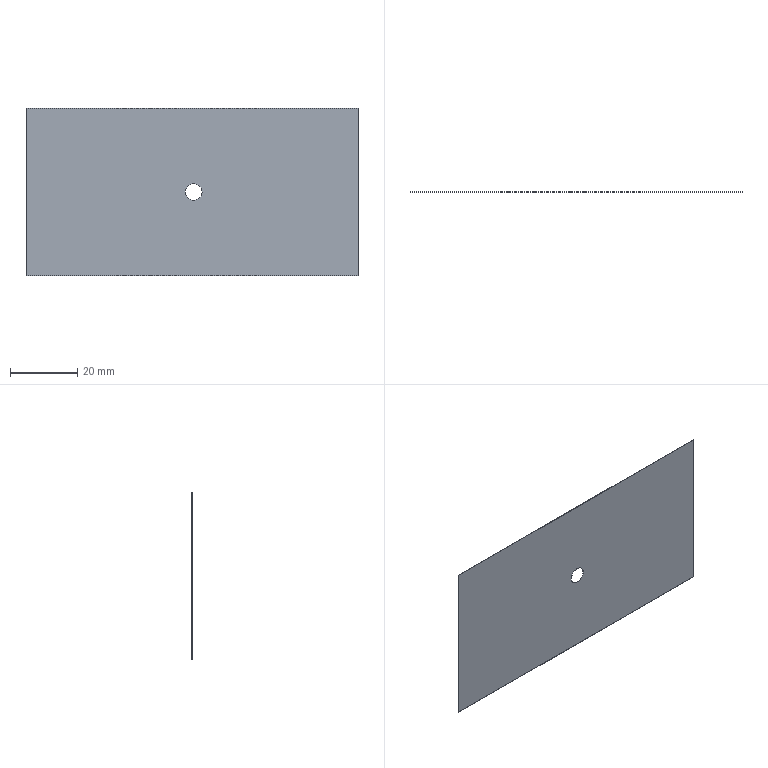Component | SolidWorks | WashingLabel100-50-1 | 1 solid | 8 faces | box 99 x 0.1 x 50 mm | volume 493 mm3 | plane 6 | cylinder 2 | commonest cylinder face diameters 5 x2 | material Zoltek Panex 33
build123d program:
from build123d import *

# Parameters (mm, degrees)
SKETCH1_W           = 50
SKETCH1_H           = 100
BOSS_EXTRUDE1_DEPTH = 0.1
SKETCH2_R           = 2.5
CUT_EXTRUDE1_DEPTH  = 10
BENDRADIUSRELIEF_BY = 1


with BuildPart() as part:
    # Sketch1 → Boss-Extrude1 (new body)
    with BuildSketch(Plane(origin=(0, 0, 0), x_dir=(1, 0, 0), z_dir=(0, 1, 0))):
        Rectangle(SKETCH1_W, SKETCH1_H)
    extrude(amount=BOSS_EXTRUDE1_DEPTH)

    # Sketch2 → Cut-Extrude1 (cut)
    with BuildSketch(Plane(origin=(0, 0.1, 0), x_dir=(1, 0, 0), z_dir=(0, 1, 0))):
        with Locations(Location((0, 0, 0), (0, 0, 270))):
            Circle(SKETCH2_R)
    extrude(amount=-CUT_EXTRUDE1_DEPTH, mode=Mode.SUBTRACT)

    # BendRadiusRelief: a face moved inward by 1.0
    extrude(part.faces().sort_by_distance((0, 0.05, -50))[0], amount=BENDRADIUSRELIEF_BY, dir=(0, 0, 1), mode=Mode.SUBTRACT)


solid = part.part

# Placed as in the assembly
solid = solid.moved(Location((12, 0, 0), (0, -90, 0)))
STEP:
#1=COLOUR_RGB('',0.7922,0.8196,0.9333);
#2=FILL_AREA_STYLE_COLOUR('',#1);
#3=FILL_AREA_STYLE('',(#2));
#4=SURFACE_STYLE_FILL_AREA(#3);
#5=SURFACE_SIDE_STYLE('',(#4));
#6=SURFACE_STYLE_USAGE(.BOTH.,#5);
#7=PRESENTATION_STYLE_ASSIGNMENT((#6));
#8=CARTESIAN_POINT('',(0.5709,0.,-0.));
#9=VERTEX_POINT('',#8);
#10=CARTESIAN_POINT('',(0.374,0.,-0.));
#11=VERTEX_POINT('',#10);
#12=CARTESIAN_POINT('',(0.4724,0.,-0.));
#13=DIRECTION('',(0.,1.,0.));
#14=DIRECTION('',(-1.,0.,-0.));
#15=AXIS2_PLACEMENT_3D('',#12,#13,#14);
#16=CIRCLE('',#15,0.09843);
#17=EDGE_CURVE('',#9,#11,#16,.T.);
#18=ORIENTED_EDGE('',*,*,#17,.F.);
#19=CARTESIAN_POINT('',(0.5709,0.003937,-0.));
#20=VERTEX_POINT('',#19);
#21=CARTESIAN_POINT('',(0.5709,-0.3898,-0.));
#22=DIRECTION('',(0.,1.,0.));
#23=VECTOR('',#22,39.37);
#24=LINE('',#21,#23);
#25=EDGE_CURVE('',#9,#20,#24,.T.);
#26=ORIENTED_EDGE('',*,*,#25,.T.);
#27=CARTESIAN_POINT('',(0.374,0.003937,-0.));
#28=VERTEX_POINT('',#27);
#29=CARTESIAN_POINT('',(0.4724,0.003937,-0.));
#30=DIRECTION('',(0.,1.,0.));
#31=DIRECTION('',(-1.,0.,-0.));
#32=AXIS2_PLACEMENT_3D('',#29,#30,#31);
#33=CIRCLE('',#32,0.09843);
#34=EDGE_CURVE('',#20,#28,#33,.T.);
#35=ORIENTED_EDGE('',*,*,#34,.T.);
#36=CARTESIAN_POINT('',(0.374,-0.3898,-0.));
#37=DIRECTION('',(0.,1.,0.));
#38=VECTOR('',#37,39.37);
#39=LINE('',#36,#38);
#40=EDGE_CURVE('',#11,#28,#39,.T.);
#41=ORIENTED_EDGE('',*,*,#40,.F.);
#42=EDGE_LOOP('',(#18,#26,#35,#41));
#43=FACE_OUTER_BOUND('',#42,.T.);
#44=CARTESIAN_POINT('',(0.4724,-0.3898,-0.));
#45=DIRECTION('',(0.,1.,0.));
#46=DIRECTION('',(-1.,0.,-0.));
#47=AXIS2_PLACEMENT_3D('',#44,#45,#46);
#48=CYLINDRICAL_SURFACE('',#47,0.09843);
#49=ADVANCED_FACE('',(#43),#48,.F.);
#50=CARTESIAN_POINT('',(-1.496,0.,0.9843));
#51=VERTEX_POINT('',#50);
#52=CARTESIAN_POINT('',(2.402,0.,0.9843));
#53=VERTEX_POINT('',#52);
#54=CARTESIAN_POINT('',(2.441,0.,0.9843));
#55=DIRECTION('',(1.,-0.,-0.));
#56=VECTOR('',#55,39.37);
#57=LINE('',#54,#56);
#58=EDGE_CURVE('',#51,#53,#57,.T.);
#59=ORIENTED_EDGE('',*,*,#58,.T.);
#60=CARTESIAN_POINT('',(2.402,0.003937,0.9843));
#61=VERTEX_POINT('',#60);
#62=CARTESIAN_POINT('',(2.402,0.003937,0.9843));
#63=DIRECTION('',(-0.,-1.,-0.));
#64=VECTOR('',#63,39.37);
#65=LINE('',#62,#64);
#66=EDGE_CURVE('',#61,#53,#65,.T.);
#67=ORIENTED_EDGE('',*,*,#66,.F.);
#68=CARTESIAN_POINT('',(-1.496,0.003937,0.9843));
#69=VERTEX_POINT('',#68);
#70=CARTESIAN_POINT('',(2.441,0.003937,0.9843));
#71=DIRECTION('',(1.,-0.,-0.));
#72=VECTOR('',#71,39.37);
#73=LINE('',#70,#72);
#74=EDGE_CURVE('',#69,#61,#73,.T.);
#75=ORIENTED_EDGE('',*,*,#74,.F.);
#76=CARTESIAN_POINT('',(-1.496,0.003937,0.9843));
#77=DIRECTION('',(-0.,-1.,-0.));
#78=VECTOR('',#77,39.37);
#79=LINE('',#76,#78);
#80=EDGE_CURVE('',#69,#51,#79,.T.);
#81=ORIENTED_EDGE('',*,*,#80,.T.);
#82=EDGE_LOOP('',(#59,#67,#75,#81));
#83=FACE_OUTER_BOUND('',#82,.T.);
#84=CARTESIAN_POINT('',(2.441,0.003937,0.9843));
#85=DIRECTION('',(-0.,0.,-1.));
#86=DIRECTION('',(-1.,0.,0.));
#87=AXIS2_PLACEMENT_3D('',#84,#85,#86);
#88=PLANE('',#87);
#89=ADVANCED_FACE('',(#83),#88,.F.);
#90=CARTESIAN_POINT('',(2.402,0.,-0.9843));
#91=VERTEX_POINT('',#90);
#92=CARTESIAN_POINT('',(2.402,0.,-0.9843));
#93=DIRECTION('',(0.,0.,-1.));
#94=VECTOR('',#93,39.37);
#95=LINE('',#92,#94);
#96=EDGE_CURVE('',#53,#91,#95,.T.);
#97=ORIENTED_EDGE('',*,*,#96,.T.);
#98=CARTESIAN_POINT('',(2.402,0.003937,-0.9843));
#99=VERTEX_POINT('',#98);
#100=CARTESIAN_POINT('',(2.402,0.003937,-0.9843));
#101=DIRECTION('',(-0.,-1.,-0.));
#102=VECTOR('',#101,39.37);
#103=LINE('',#100,#102);
#104=EDGE_CURVE('',#99,#91,#103,.T.);
#105=ORIENTED_EDGE('',*,*,#104,.F.);
#106=CARTESIAN_POINT('',(2.402,0.003937,-0.9843));
#107=DIRECTION('',(0.,0.,-1.));
#108=VECTOR('',#107,39.37);
#109=LINE('',#106,#108);
#110=EDGE_CURVE('',#61,#99,#109,.T.);
#111=ORIENTED_EDGE('',*,*,#110,.F.);
#112=ORIENTED_EDGE('',*,*,#66,.T.);
#113=EDGE_LOOP('',(#97,#105,#111,#112));
#114=FACE_OUTER_BOUND('',#113,.T.);
#115=CARTESIAN_POINT('',(2.402,0.003937,-0.9843));
#116=DIRECTION('',(-1.,0.,-0.));
#117=DIRECTION('',(-0.,-0.,1.));
#118=AXIS2_PLACEMENT_3D('',#115,#116,#117);
#119=PLANE('',#118);
#120=ADVANCED_FACE('',(#114),#119,.F.);
#121=CARTESIAN_POINT('',(-1.496,0.,-0.9843));
#122=VERTEX_POINT('',#121);
#123=CARTESIAN_POINT('',(2.441,0.,-0.9843));
#124=DIRECTION('',(-1.,0.,0.));
#125=VECTOR('',#124,39.37);
#126=LINE('',#123,#125);
#127=EDGE_CURVE('',#91,#122,#126,.T.);
#128=ORIENTED_EDGE('',*,*,#127,.T.);
#129=CARTESIAN_POINT('',(-1.496,0.003937,-0.9843));
#130=VERTEX_POINT('',#129);
#131=CARTESIAN_POINT('',(-1.496,0.003937,-0.9843));
#132=DIRECTION('',(-0.,-1.,-0.));
#133=VECTOR('',#132,39.37);
#134=LINE('',#131,#133);
#135=EDGE_CURVE('',#130,#122,#134,.T.);
#136=ORIENTED_EDGE('',*,*,#135,.F.);
#137=CARTESIAN_POINT('',(2.441,0.003937,-0.9843));
#138=DIRECTION('',(-1.,0.,0.));
#139=VECTOR('',#138,39.37);
#140=LINE('',#137,#139);
#141=EDGE_CURVE('',#99,#130,#140,.T.);
#142=ORIENTED_EDGE('',*,*,#141,.F.);
#143=ORIENTED_EDGE('',*,*,#104,.T.);
#144=EDGE_LOOP('',(#128,#136,#142,#143));
#145=FACE_OUTER_BOUND('',#144,.T.);
#146=CARTESIAN_POINT('',(2.441,0.003937,-0.9843));
#147=DIRECTION('',(0.,-0.,1.));
#148=DIRECTION('',(1.,-0.,-0.));
#149=AXIS2_PLACEMENT_3D('',#146,#147,#148);
#150=PLANE('',#149);
#151=ADVANCED_FACE('',(#145),#150,.F.);
#152=CARTESIAN_POINT('',(-1.496,0.,-0.9843));
#153=DIRECTION('',(-0.,-0.,1.));
#154=VECTOR('',#153,39.37);
#155=LINE('',#152,#154);
#156=EDGE_CURVE('',#122,#51,#155,.T.);
#157=ORIENTED_EDGE('',*,*,#156,.T.);
#158=ORIENTED_EDGE('',*,*,#80,.F.);
#159=CARTESIAN_POINT('',(-1.496,0.003937,-0.9843));
#160=DIRECTION('',(-0.,-0.,1.));
#161=VECTOR('',#160,39.37);
#162=LINE('',#159,#161);
#163=EDGE_CURVE('',#130,#69,#162,.T.);
#164=ORIENTED_EDGE('',*,*,#163,.F.);
#165=ORIENTED_EDGE('',*,*,#135,.T.);
#166=EDGE_LOOP('',(#157,#158,#164,#165));
#167=FACE_OUTER_BOUND('',#166,.T.);
#168=CARTESIAN_POINT('',(-1.496,0.003937,-0.9843));
#169=DIRECTION('',(1.,-0.,0.));
#170=DIRECTION('',(0.,0.,-1.));
#171=AXIS2_PLACEMENT_3D('',#168,#169,#170);
#172=PLANE('',#171);
#173=ADVANCED_FACE('',(#167),#172,.F.);
#174=CARTESIAN_POINT('',(0.4724,0.003937,-0.));
#175=DIRECTION('',(0.,1.,0.));
#176=DIRECTION('',(-1.,0.,-0.));
#177=AXIS2_PLACEMENT_3D('',#174,#175,#176);
#178=CIRCLE('',#177,0.09843);
#179=EDGE_CURVE('',#28,#20,#178,.T.);
#180=ORIENTED_EDGE('',*,*,#179,.F.);
#181=ORIENTED_EDGE('',*,*,#34,.F.);
#182=EDGE_LOOP('',(#180,#181));
#183=FACE_BOUND('',#182,.T.);
#184=ORIENTED_EDGE('',*,*,#74,.T.);
#185=ORIENTED_EDGE('',*,*,#110,.T.);
#186=ORIENTED_EDGE('',*,*,#141,.T.);
#187=ORIENTED_EDGE('',*,*,#163,.T.);
#188=EDGE_LOOP('',(#184,#185,#186,#187));
#189=FACE_OUTER_BOUND('',#188,.T.);
#190=CARTESIAN_POINT('',(0.4724,0.003937,-0.));
#191=DIRECTION('',(0.,1.,0.));
#192=DIRECTION('',(-1.,0.,-0.));
#193=AXIS2_PLACEMENT_3D('',#190,#191,#192);
#194=PLANE('',#193);
#195=ADVANCED_FACE('',(#183,#189),#194,.T.);
#196=CARTESIAN_POINT('',(0.4724,0.,-0.));
#197=DIRECTION('',(0.,1.,0.));
#198=DIRECTION('',(-1.,0.,-0.));
#199=AXIS2_PLACEMENT_3D('',#196,#197,#198);
#200=CIRCLE('',#199,0.09843);
#201=EDGE_CURVE('',#11,#9,#200,.T.);
#202=ORIENTED_EDGE('',*,*,#201,.T.);
#203=ORIENTED_EDGE('',*,*,#17,.T.);
#204=EDGE_LOOP('',(#202,#203));
#205=FACE_BOUND('',#204,.T.);
#206=ORIENTED_EDGE('',*,*,#58,.F.);
#207=ORIENTED_EDGE('',*,*,#156,.F.);
#208=ORIENTED_EDGE('',*,*,#127,.F.);
#209=ORIENTED_EDGE('',*,*,#96,.F.);
#210=EDGE_LOOP('',(#206,#207,#208,#209));
#211=FACE_OUTER_BOUND('',#210,.T.);
#212=CARTESIAN_POINT('',(0.4724,0.,-0.));
#213=DIRECTION('',(0.,1.,0.));
#214=DIRECTION('',(-1.,0.,-0.));
#215=AXIS2_PLACEMENT_3D('',#212,#213,#214);
#216=PLANE('',#215);
#217=ADVANCED_FACE('',(#205,#211),#216,.F.);
#218=ORIENTED_EDGE('',*,*,#25,.F.);
#219=ORIENTED_EDGE('',*,*,#201,.F.);
#220=ORIENTED_EDGE('',*,*,#40,.T.);
#221=ORIENTED_EDGE('',*,*,#179,.T.);
#222=EDGE_LOOP('',(#218,#219,#220,#221));
#223=FACE_OUTER_BOUND('',#222,.T.);
#224=CARTESIAN_POINT('',(0.4724,-0.3898,-0.));
#225=DIRECTION('',(0.,1.,0.));
#226=DIRECTION('',(-1.,0.,-0.));
#227=AXIS2_PLACEMENT_3D('',#224,#225,#226);
#228=CYLINDRICAL_SURFACE('',#227,0.09843);
#229=ADVANCED_FACE('',(#223),#228,.F.);
#230=CLOSED_SHELL('',(#49,#89,#120,#151,#173,#195,#217,#229));
#231=MANIFOLD_SOLID_BREP('',#230);
#232=STYLED_ITEM('',(#7),#231);
#233=PRESENTATION_LAYER_ASSIGNMENT('','',(#232));
#234=(LENGTH_UNIT()NAMED_UNIT(*)SI_UNIT($,.METRE.));
#235=LENGTH_MEASURE_WITH_UNIT(LENGTH_MEASURE(0.0254),#234);
#236=DIMENSIONAL_EXPONENTS(1.,0.,0.,0.,0.,0.,0.);
#237=(CONVERSION_BASED_UNIT('',#235)LENGTH_UNIT()NAMED_UNIT(#236));
#238=UNCERTAINTY_MEASURE_WITH_UNIT(LENGTH_MEASURE(0.00001),#237,'','');
#239=(NAMED_UNIT(*)PLANE_ANGLE_UNIT()SI_UNIT($,.RADIAN.));
#240=(NAMED_UNIT(*)SI_UNIT($,.STERADIAN.)SOLID_ANGLE_UNIT());
#241=(GEOMETRIC_REPRESENTATION_CONTEXT(3)GLOBAL_UNCERTAINTY_ASSIGNED_CONTEXT((#238))GLOBAL_UNIT_ASSIGNED_CONTEXT((#237,#239,#240))REPRESENTATION_CONTEXT('',''));
#242=MECHANICAL_DESIGN_GEOMETRIC_PRESENTATION_REPRESENTATION('',(#232),#241);
#243=CARTESIAN_POINT('',(0.,0.,0.));
#244=DIRECTION('',(0.,0.,1.));
#245=DIRECTION('',(1.,0.,0.));
#246=AXIS2_PLACEMENT_3D('',#243,#244,#245);
#247=(LENGTH_UNIT()NAMED_UNIT(*)SI_UNIT($,.METRE.));
#248=LENGTH_MEASURE_WITH_UNIT(LENGTH_MEASURE(0.0254),#247);
#249=DIMENSIONAL_EXPONENTS(1.,0.,0.,0.,0.,0.,0.);
#250=(CONVERSION_BASED_UNIT('',#248)LENGTH_UNIT()NAMED_UNIT(#249));
#251=UNCERTAINTY_MEASURE_WITH_UNIT(LENGTH_MEASURE(0.00001),#250,'','');
#252=(NAMED_UNIT(*)PLANE_ANGLE_UNIT()SI_UNIT($,.RADIAN.));
#253=(NAMED_UNIT(*)SI_UNIT($,.STERADIAN.)SOLID_ANGLE_UNIT());
#254=(GEOMETRIC_REPRESENTATION_CONTEXT(3)GLOBAL_UNCERTAINTY_ASSIGNED_CONTEXT((#251))GLOBAL_UNIT_ASSIGNED_CONTEXT((#250,#252,#253))REPRESENTATION_CONTEXT('',''));
#255=ADVANCED_BREP_SHAPE_REPRESENTATION('',(#231,#246),#254);